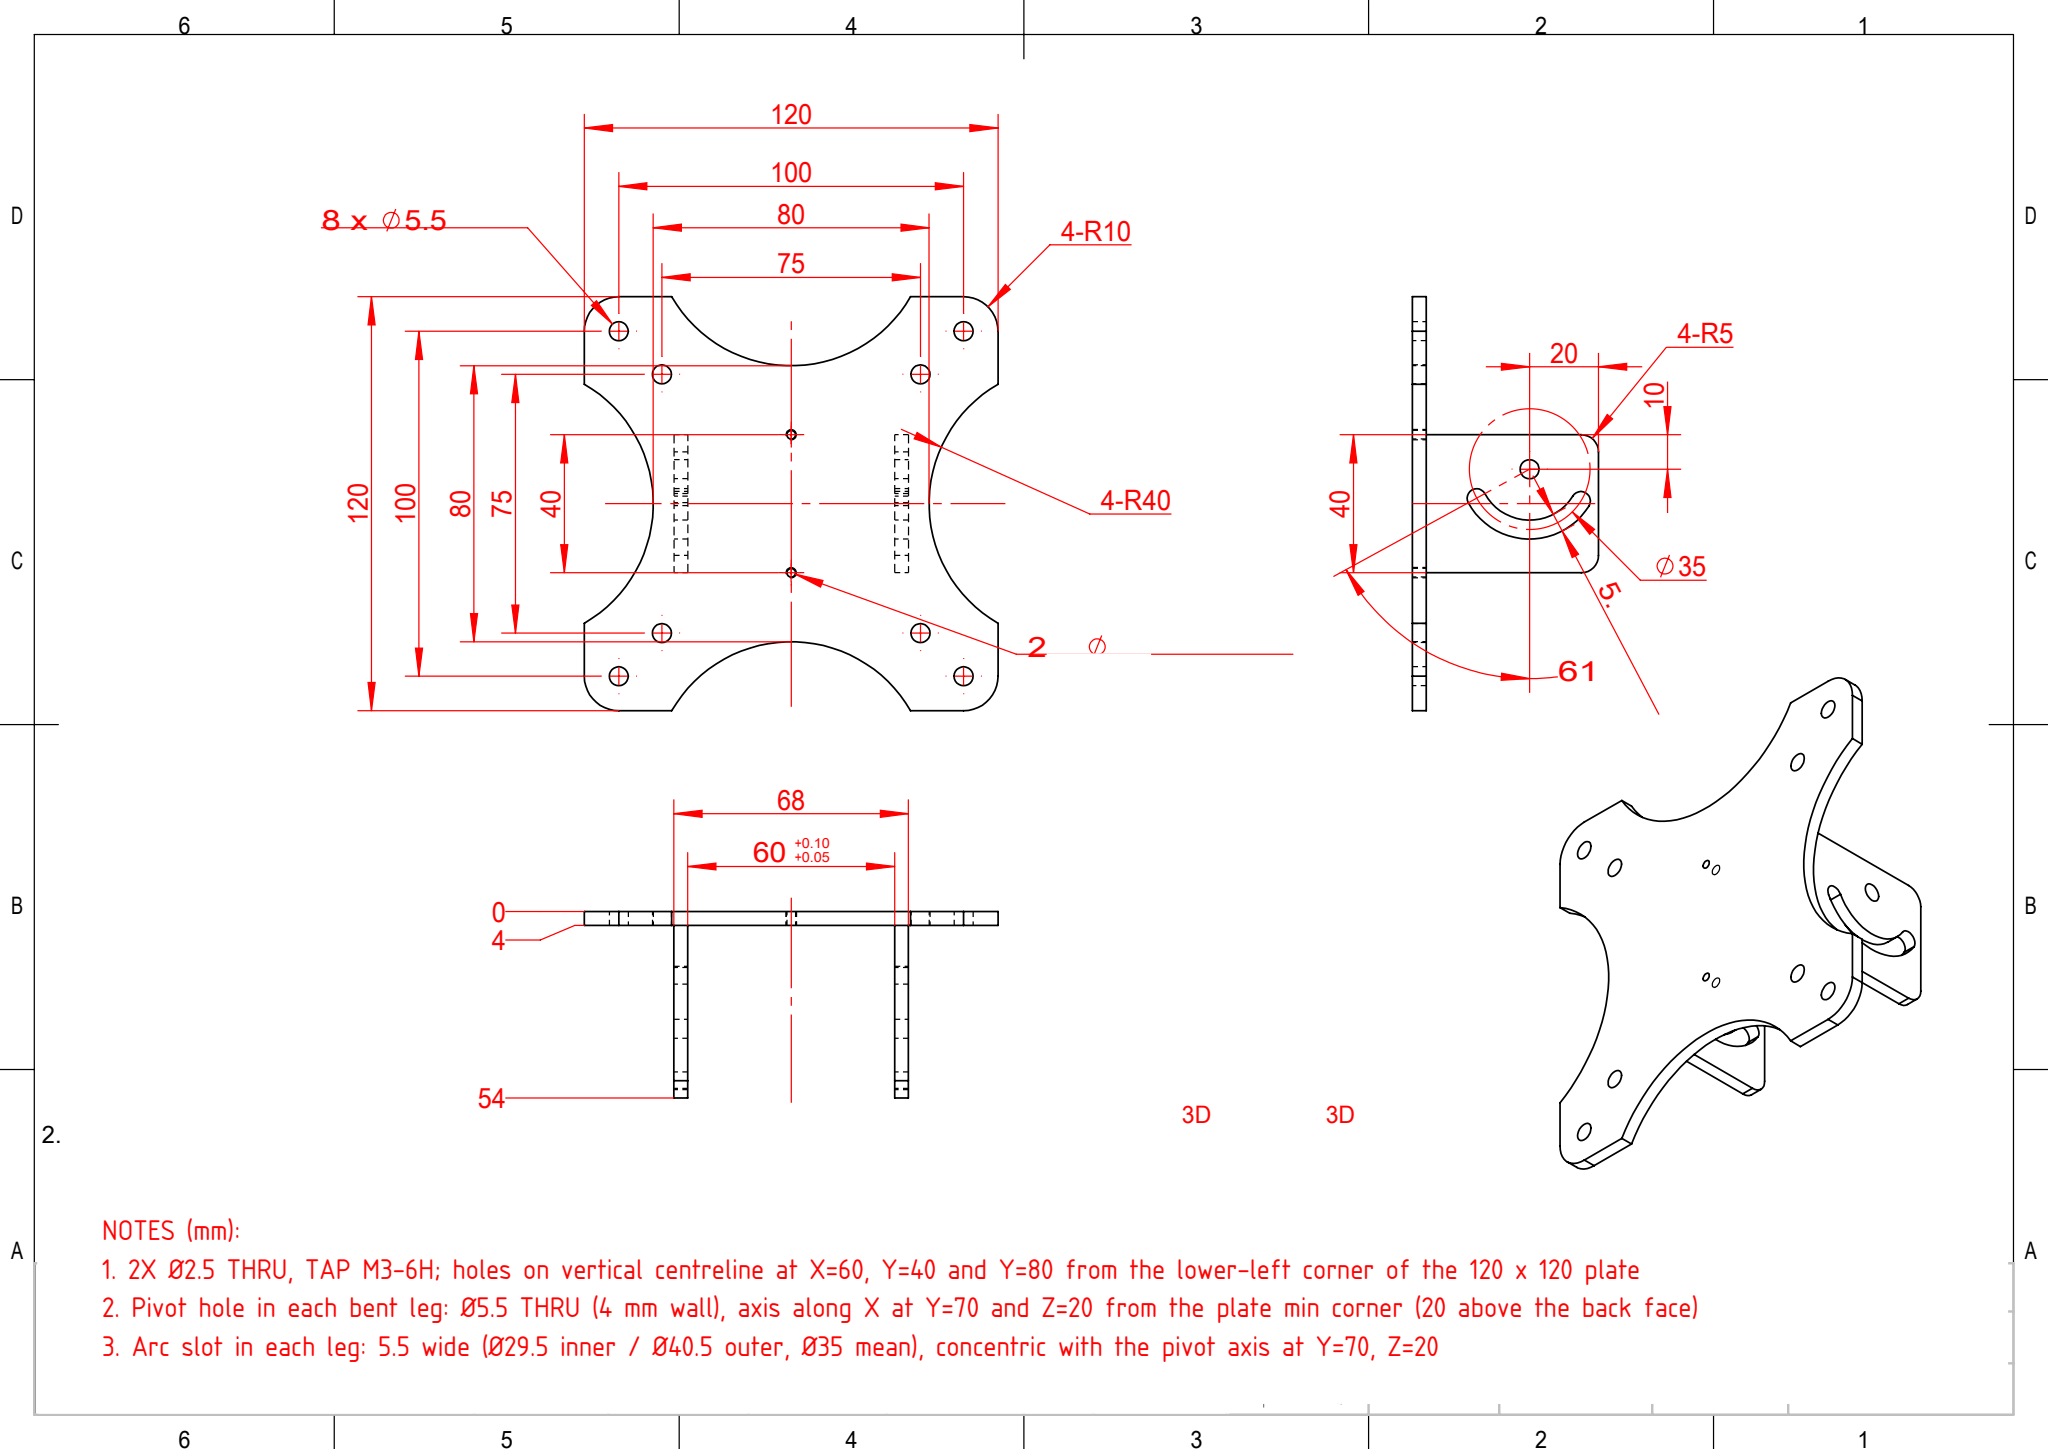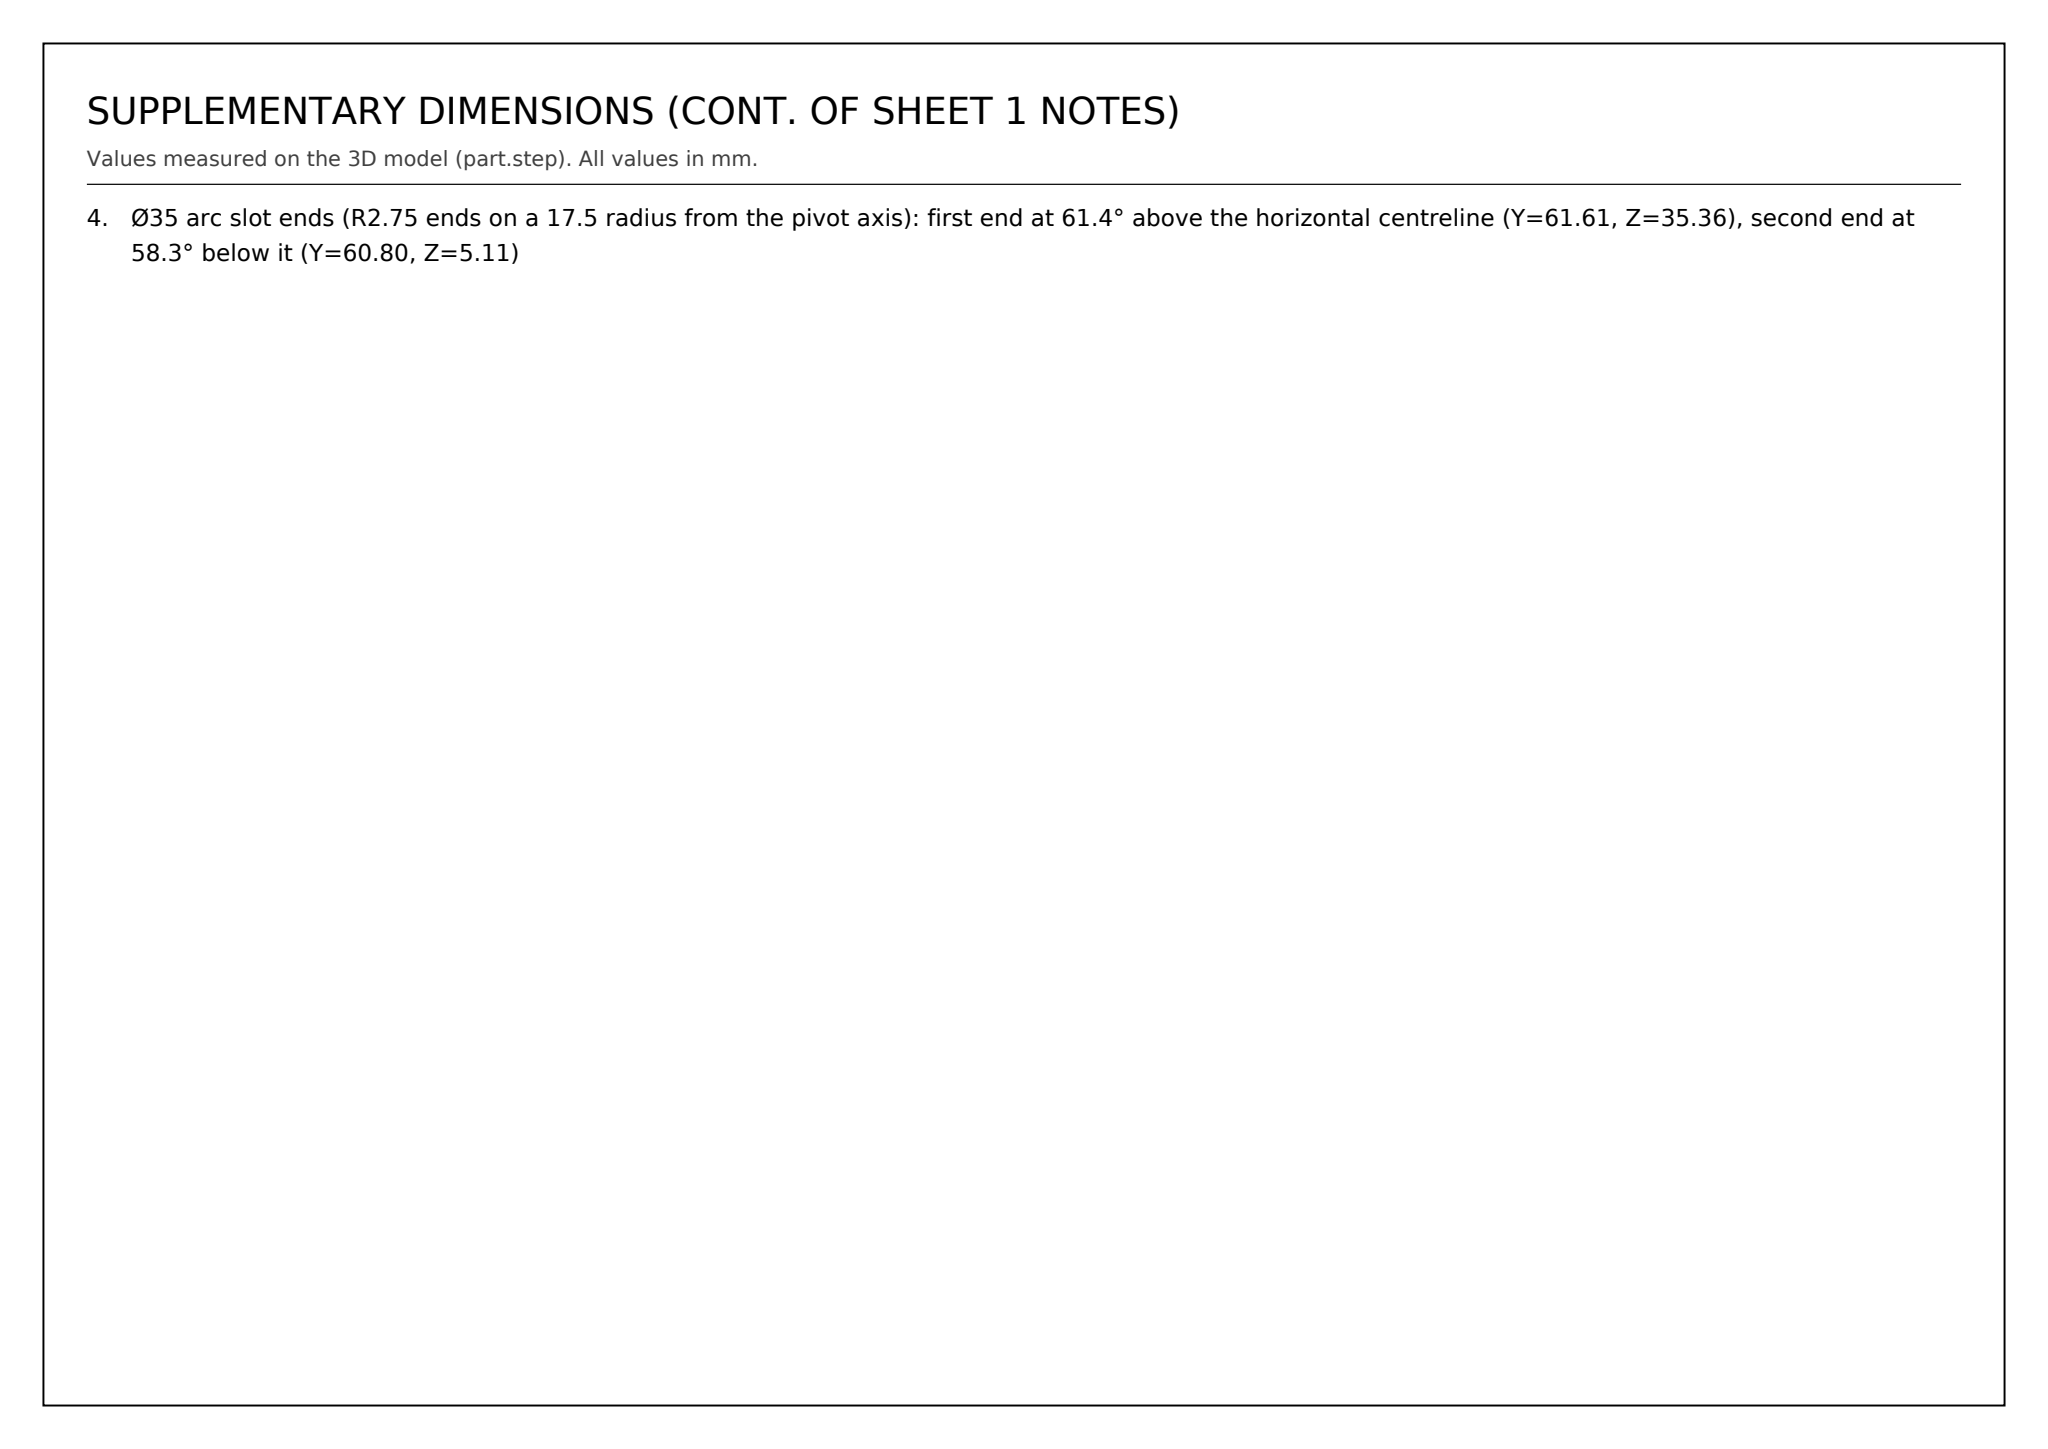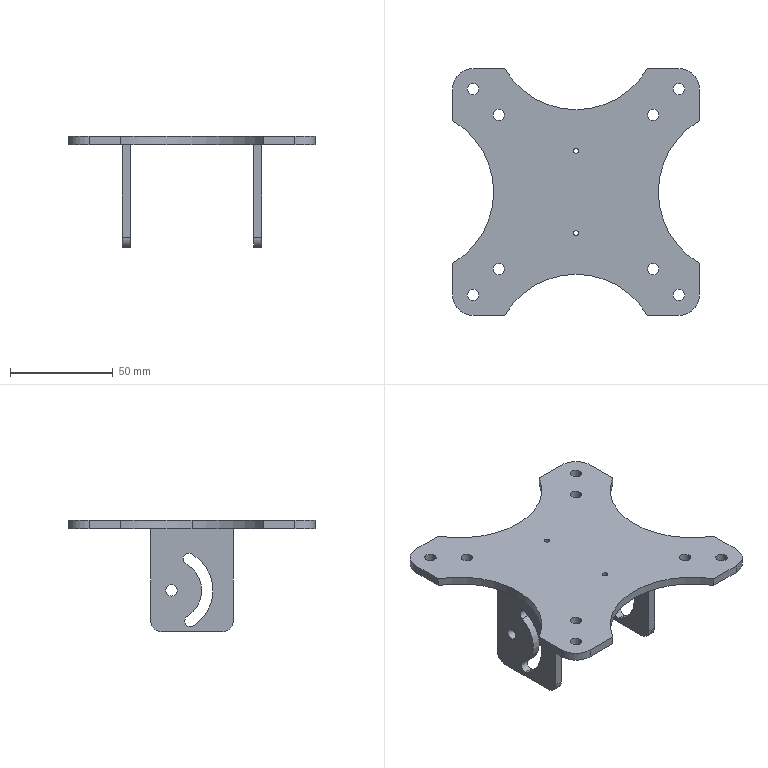Part | SolidWorks | mm | 1 solid | 67 faces | box 120 x 120 x 54 mm | volume 54660 mm3 | cylinder 47 | plane 20 | commonest cylinder face diameters 5.5 x22 80 x5 2.5 x4 5.503 x4 20 x4 10 x4 29.5 x2 40.5 x2
Drawing notes:
2X Ø2.5 THRU, TAP M3-6H; holes on vertical centreline at X=60, Y=40 and Y=80 from the lower-left corner of the 120 x 120 plate | from the solid: cylinders [2.5,"z",[60.0,40.0],len 4.0] and [2.5,"z",[60.0,80.0],len 4.0]
Pivot hole in each bent leg: Ø5.5 THRU (4 mm wall), axis along X at Y=70 and Z=20 from the plate min corner (20 above the back face) | from the solid: cylinders [5.5,"x",[null,70.0,20.0],len 4.0]
Arc slot in each leg: 5.5 wide (Ø29.5 inner / Ø40.5 outer, Ø35 mean), concentric with the pivot axis at Y=70, Z=20 | from the solid: cylinders [29.5,"x",[null,70.0,20.0]] and [40.5,"x",[null,70.0,20.0]]
Ø35 arc slot ends (R2.75 ends on a 17.5 radius from the pivot axis): first end at 61.4° above the horizontal centreline (Y=61.61, Z=35.36), second end at 58.3° below it (Y=60.80, Z=5.11) | from the solid: cylinders [5.5,"x",[null,61.61,35.36]] and [5.503,"x",[null,60.8,5.11]]